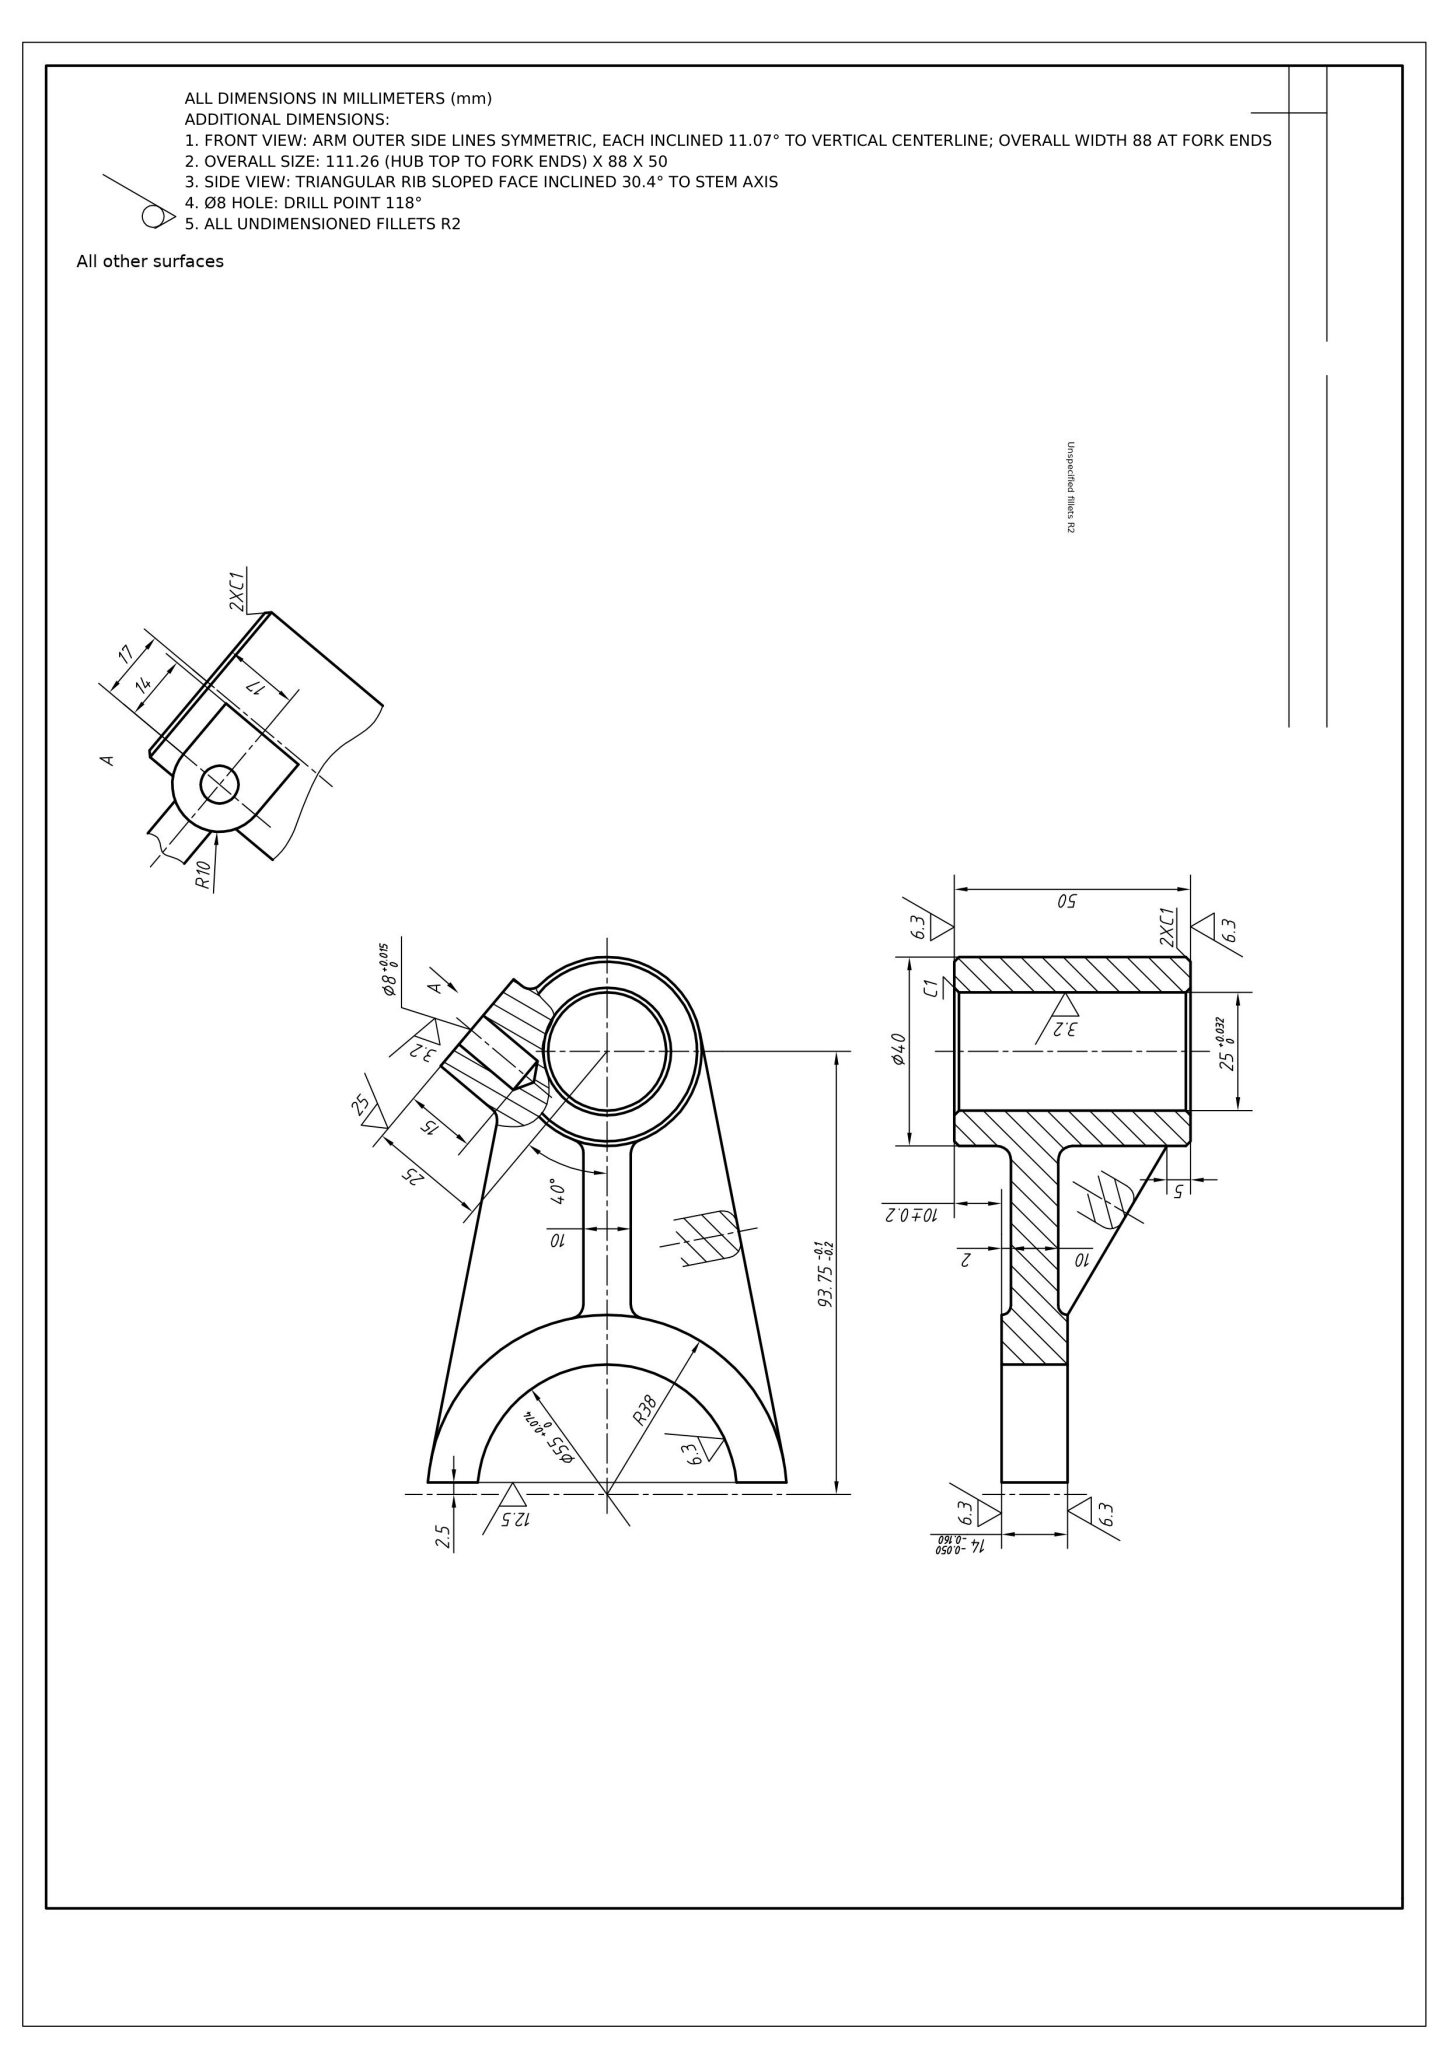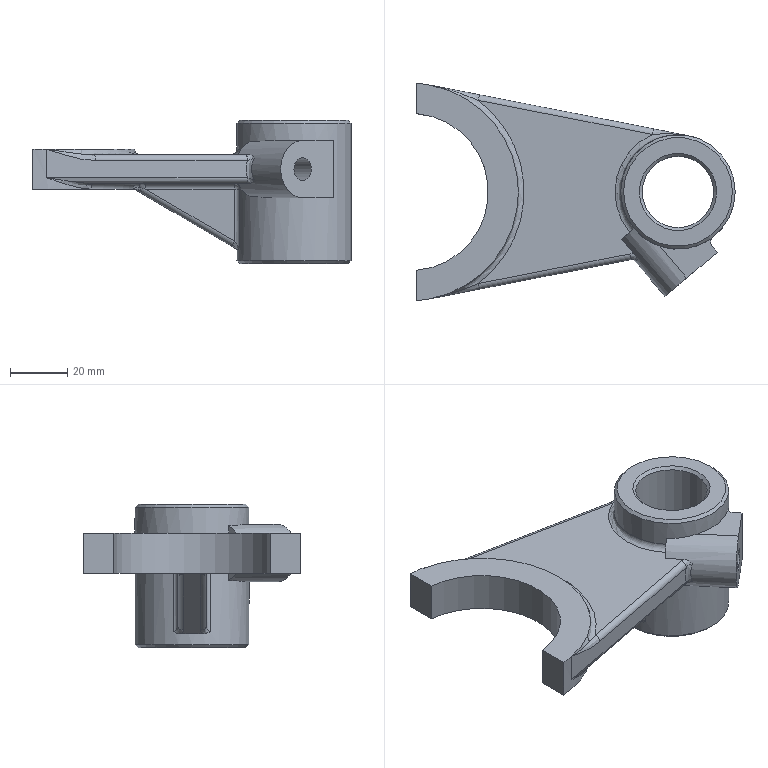Part | NX | mm | 1 solid | 71 faces | box 111.25 x 75.84 x 50 mm | volume 87573 mm3 | plane 20 | cylinder 19 | spline 17 | torus 6 | cone 5 | sphere 4 | commonest cylinder face diameters 4 x12 76 x2 40 x1 55 x1 20 x1 25 x1 8 x1